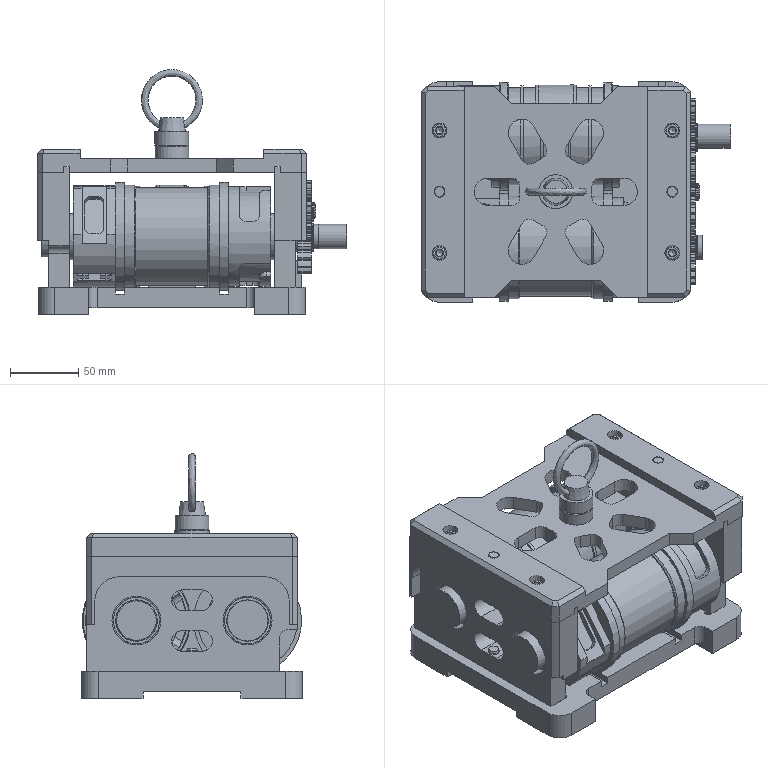Assembly | NX | mm | 31 component files | 111 solids | 1499 faces | box 227.5 x 162 x 180 mm | volume 2309783 mm3 | plane 559 | cylinder 357 | other 200 | spline 152 | cone 131 | sphere 76 | torus 24 | commonest cylinder face diameters 10 x42 43.75 x40 12 x28 8 x20 5.795 x16 33.45 x16 34 x12 5 x12
Bill of materials:
unnamed part 1 | 1 |  | Rectangular plate with rounded corners, a large central through-hole, and shallow straight channels running across the top face.
unnamed part 2 | 1 |  | Pin with a ring handle: a toroidal ring attached to a tapered head, above a wider cylindrical collar and a smaller cylindrical shank with a chamfered tip.
unnamed part 3 | 1 |  | Flat spur-type gear with about 16 straight teeth and a plain round center bore.
unnamed part 4 | 1 |  | Rectangular plate-like block with two large round through-holes, two obround slots, a small cylindrical boss with a groove, and a ledge along the top edge with small holes.
unnamed part 5 | 2 |  | Flat spur-type gear with about 20 straight teeth and a round bore with a single rectangular keyway.
unnamed part 6 | 2 |  | Thin flat open ring with two lugs, each with a small hole, on either side of a radial gap. The shape matches an external-style retaining ring.
unnamed part 7 | 1 |  | Elongated cylindrical housing-like body with stepped shaft ends, raised circumferential bands, a rectangular block near one end with a round hole, and several slots and notches.
unnamed part 8 | 1 |  | Rectangular plate with six obround slots arranged radially around a central raised boss with a small hole, waisted chamfered side cutouts, and edge holes along a stepped rail.
GB-T119.1-2000,8x32 | 4 |  | Parallel Pin, GB-T 119.1-2000,8x32
unnamed part 9 | 1 |  | Thin flat open ring with two lugs, each with a small hole, beside an angled gap. The shape matches a retaining ring.
GB-T292_C-1994,71806_C | 4 |  | Thin-section annular assembly that looks like a radial ball bearing: a plain outer ring and a plain inner ring sharing one axis, with a single row of spherical balls spaced evenly in the annular gap between them. No seals or shields cover the open faces. The axial width is small compared with the diameter.
unnamed part 10 | 2 |  | Solid obround (stadium-shaped) prism: a straight extrusion of a rectangle with two semicircular ends.
unnamed part 11 | 1 |  | Elongated cylindrical housing-like body with stepped shaft ends, raised circumferential flanges, a square block near one end, and slots and notches.
unnamed part 12 | 1 |  | Rectangular plate-like block with two large round through-holes, two obround slots between them, small holes along the top edge, and a notched corner.
GB-T70.1-2000,M6x20 | 8 |  | Hexagon Socket Head Cap Screw, GB-T 70.1-2000,M6x20
Mates:
1. fix | Base_Plate 1 component
2. touch align | Left_Side_Plate 1 face | Base_Plate 1 face
3. touch align | Left_Side_Plate 1 face | Base_Plate 1 face
4. touch align | Left_Side_Plate 1 face | Base_Plate 1 face
5. touch align | Right_Side_Plate 1 face | Base_Plate 1 face
6. touch align | Right_Side_Plate 1 face | Base_Plate 1 face
7. touch align | Right_Side_Plate 1 face | Base_Plate 1 face
8. touch align | Top_Cover 1 face | Left_Side_Plate 1 face
9. concentric | Top_Cover 1 edge | Left_Side_Plate 1 edge
10. concentric | GB-T292_C-1994_71806_C 1 edge | Right_Side_Plate 1 edge
11. concentric | GB-T292_C-1994_71806_C 2 edge | Right_Side_Plate 1 edge
12. concentric | GB-T292_C-1994_71806_C 3 edge | Left_Side_Plate 1 edge
13. concentric | GB-T292_C-1994_71806_C 4 edge | Left_Side_Plate 1 edge
14. concentric | Drive_Shaft 1 edge | GB-T292_C-1994_71806_C 1 edge
15. concentric | Driven_Shaft 1 edge | GB-T292_C-1994_71806_C 2 edge
16. concentric | Gear_1 1 edge | Driven_Shaft 1 edge
17. concentric | Gear_1 2 edge | Drive_Shaft 1 edge
18. touch align | Idler_Gear 1 face | Right_Side_Plate 1 face
19. touch align | Idler_Gear 1 face | Gear_1 2 face
20. concentric | Circlip_Shaft_A10 1 edge | Right_Side_Plate 1 edge
21. concentric | Circlip_Shaft_A16 2 edge | Driven_Shaft 1 edge
22. concentric | Circlip_Shaft_A16 1 edge | Drive_Shaft 1 edge
23. touch align | Key_A 1 face | Gear_1 1 face
24. touch align | Key_A 1 face | Gear_1 1 face
25. touch align | Key_A 1 face | Gear_1 1 face
26. touch align | Key_A 2 face | Gear_1 2 face
27. touch align | Key_A 2 face | Gear_1 2 face
28. touch align | Key_A 2 face | Gear_1 2 face
29. concentric | Lifting_Eye_M10 1 edge | Top_Cover 1 edge
30. concentric | GB-T70_1-2000_M6x20 8 edge | Top_Cover 1 edge
31. concentric | GB-T70_1-2000_M6x20 4 edge | Top_Cover 1 edge
32. concentric | GB-T70_1-2000_M6x20 7 edge | Top_Cover 1 edge
33. concentric | GB-T70_1-2000_M6x20 2 edge | Top_Cover 1 edge
34. concentric | GB-T70_1-2000_M6x20 1 edge | Base_Plate 1 edge
35. concentric | GB-T70_1-2000_M6x20 6 edge | Base_Plate 1 edge
36. concentric | GB-T70_1-2000_M6x20 5 edge | Base_Plate 1 edge
37. concentric | GB-T70_1-2000_M6x20 3 edge | Base_Plate 1 edge
38. concentric | GB-T119_1-2000_8x32 4 edge | Base_Plate 1 edge
39. concentric | GB-T119_1-2000_8x32 3 edge | Base_Plate 1 edge
40. concentric | GB-T119_1-2000_8x32 2 edge | Top_Cover 1 edge
41. concentric | GB-T119_1-2000_8x32 1 edge | Top_Cover 1 edge